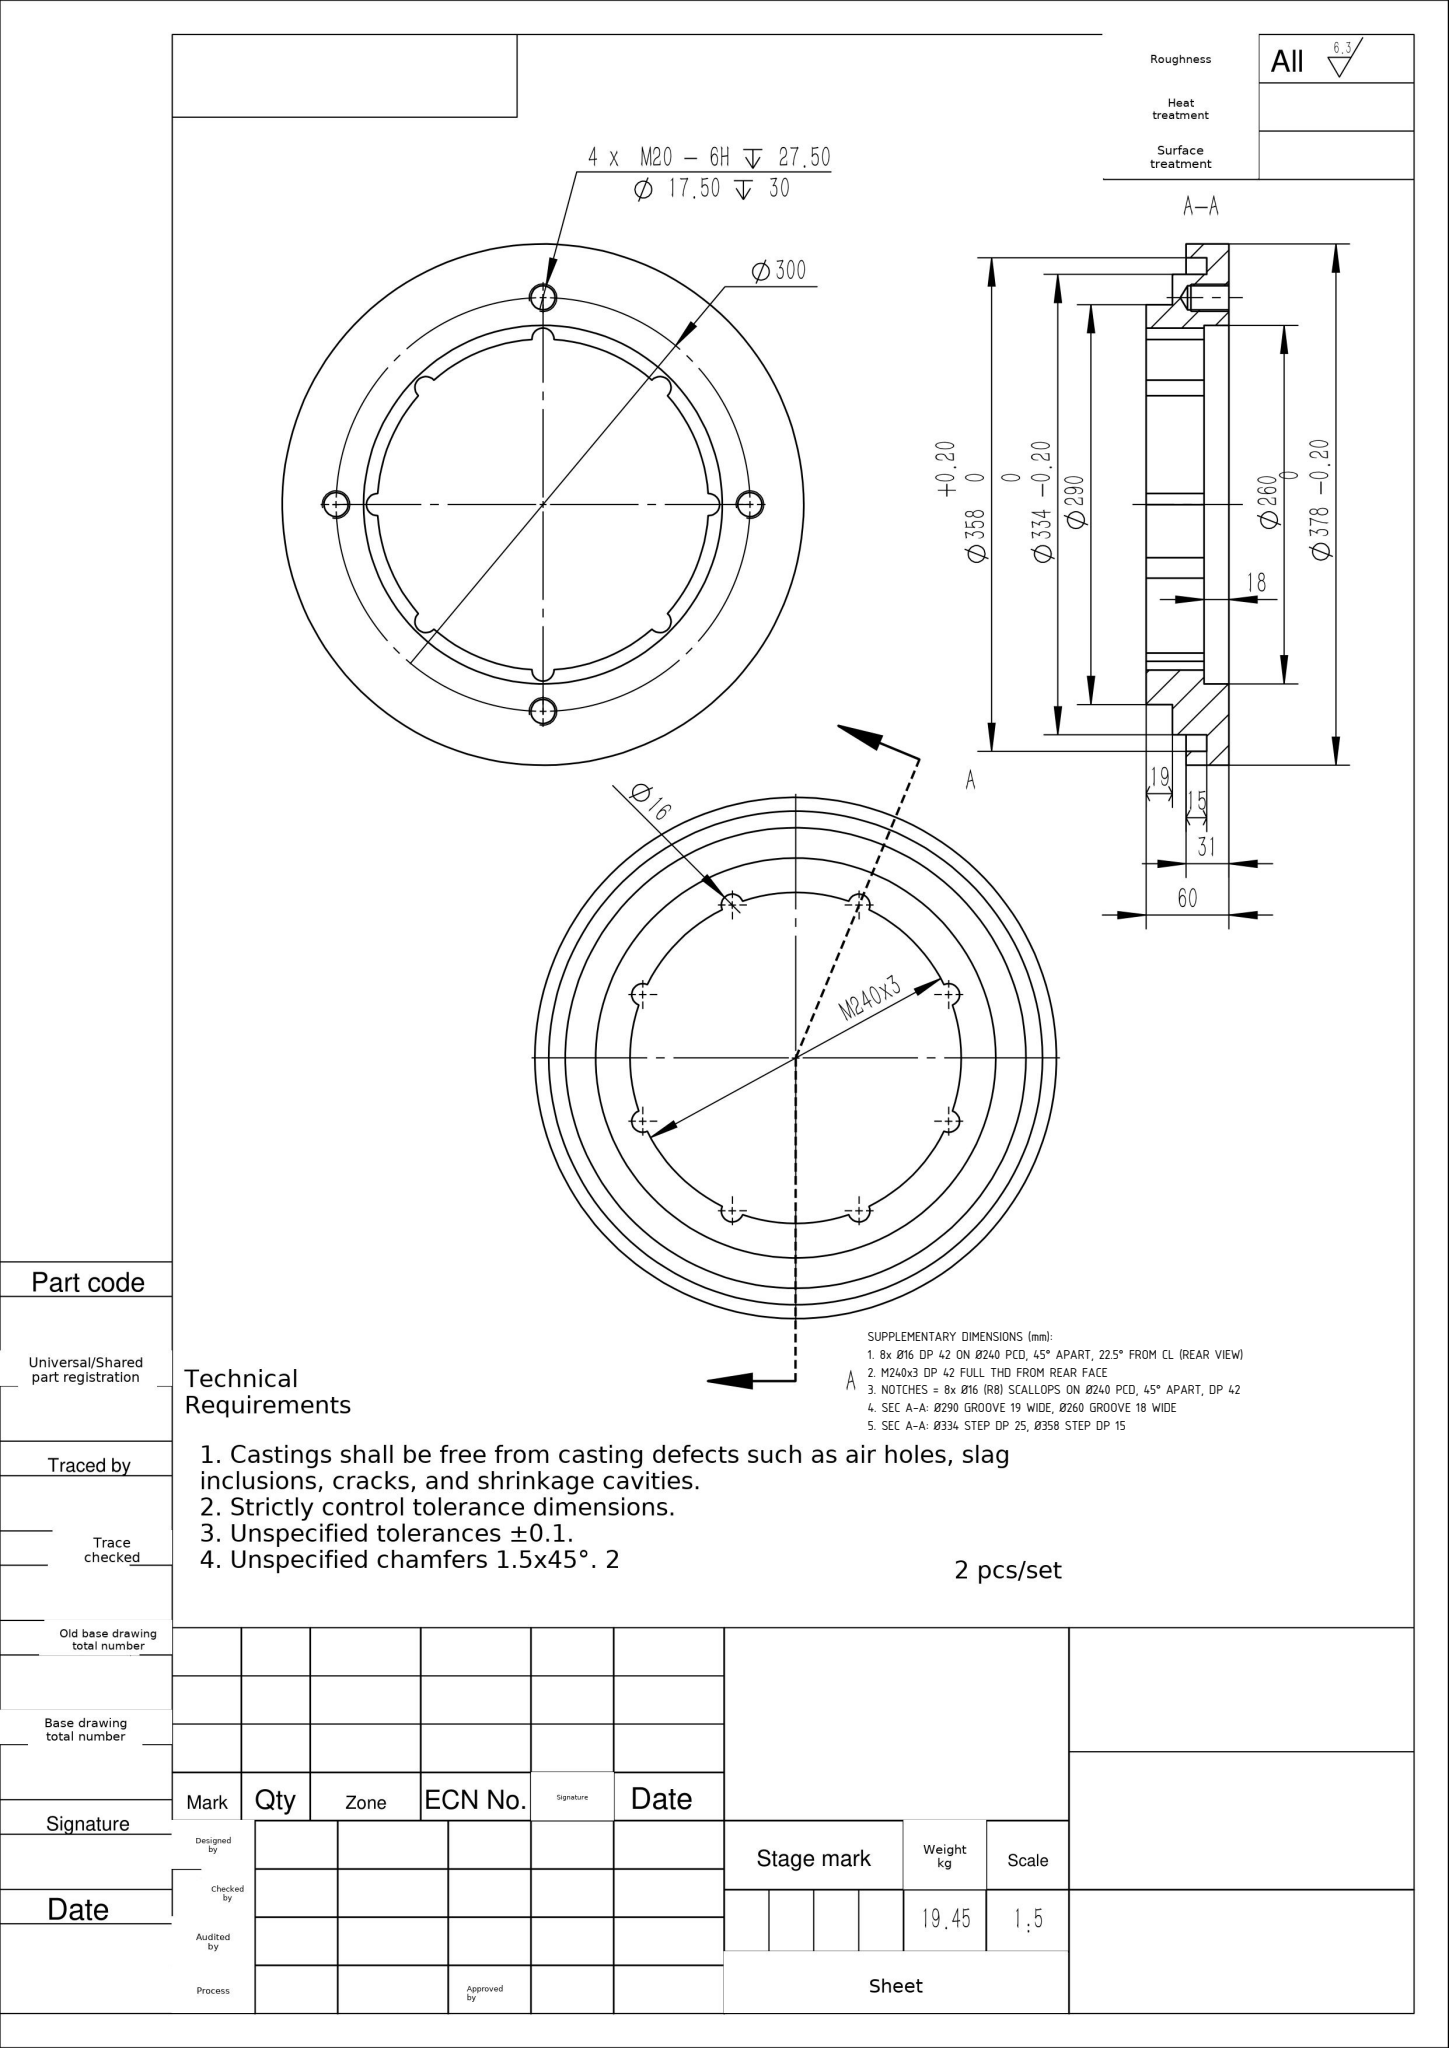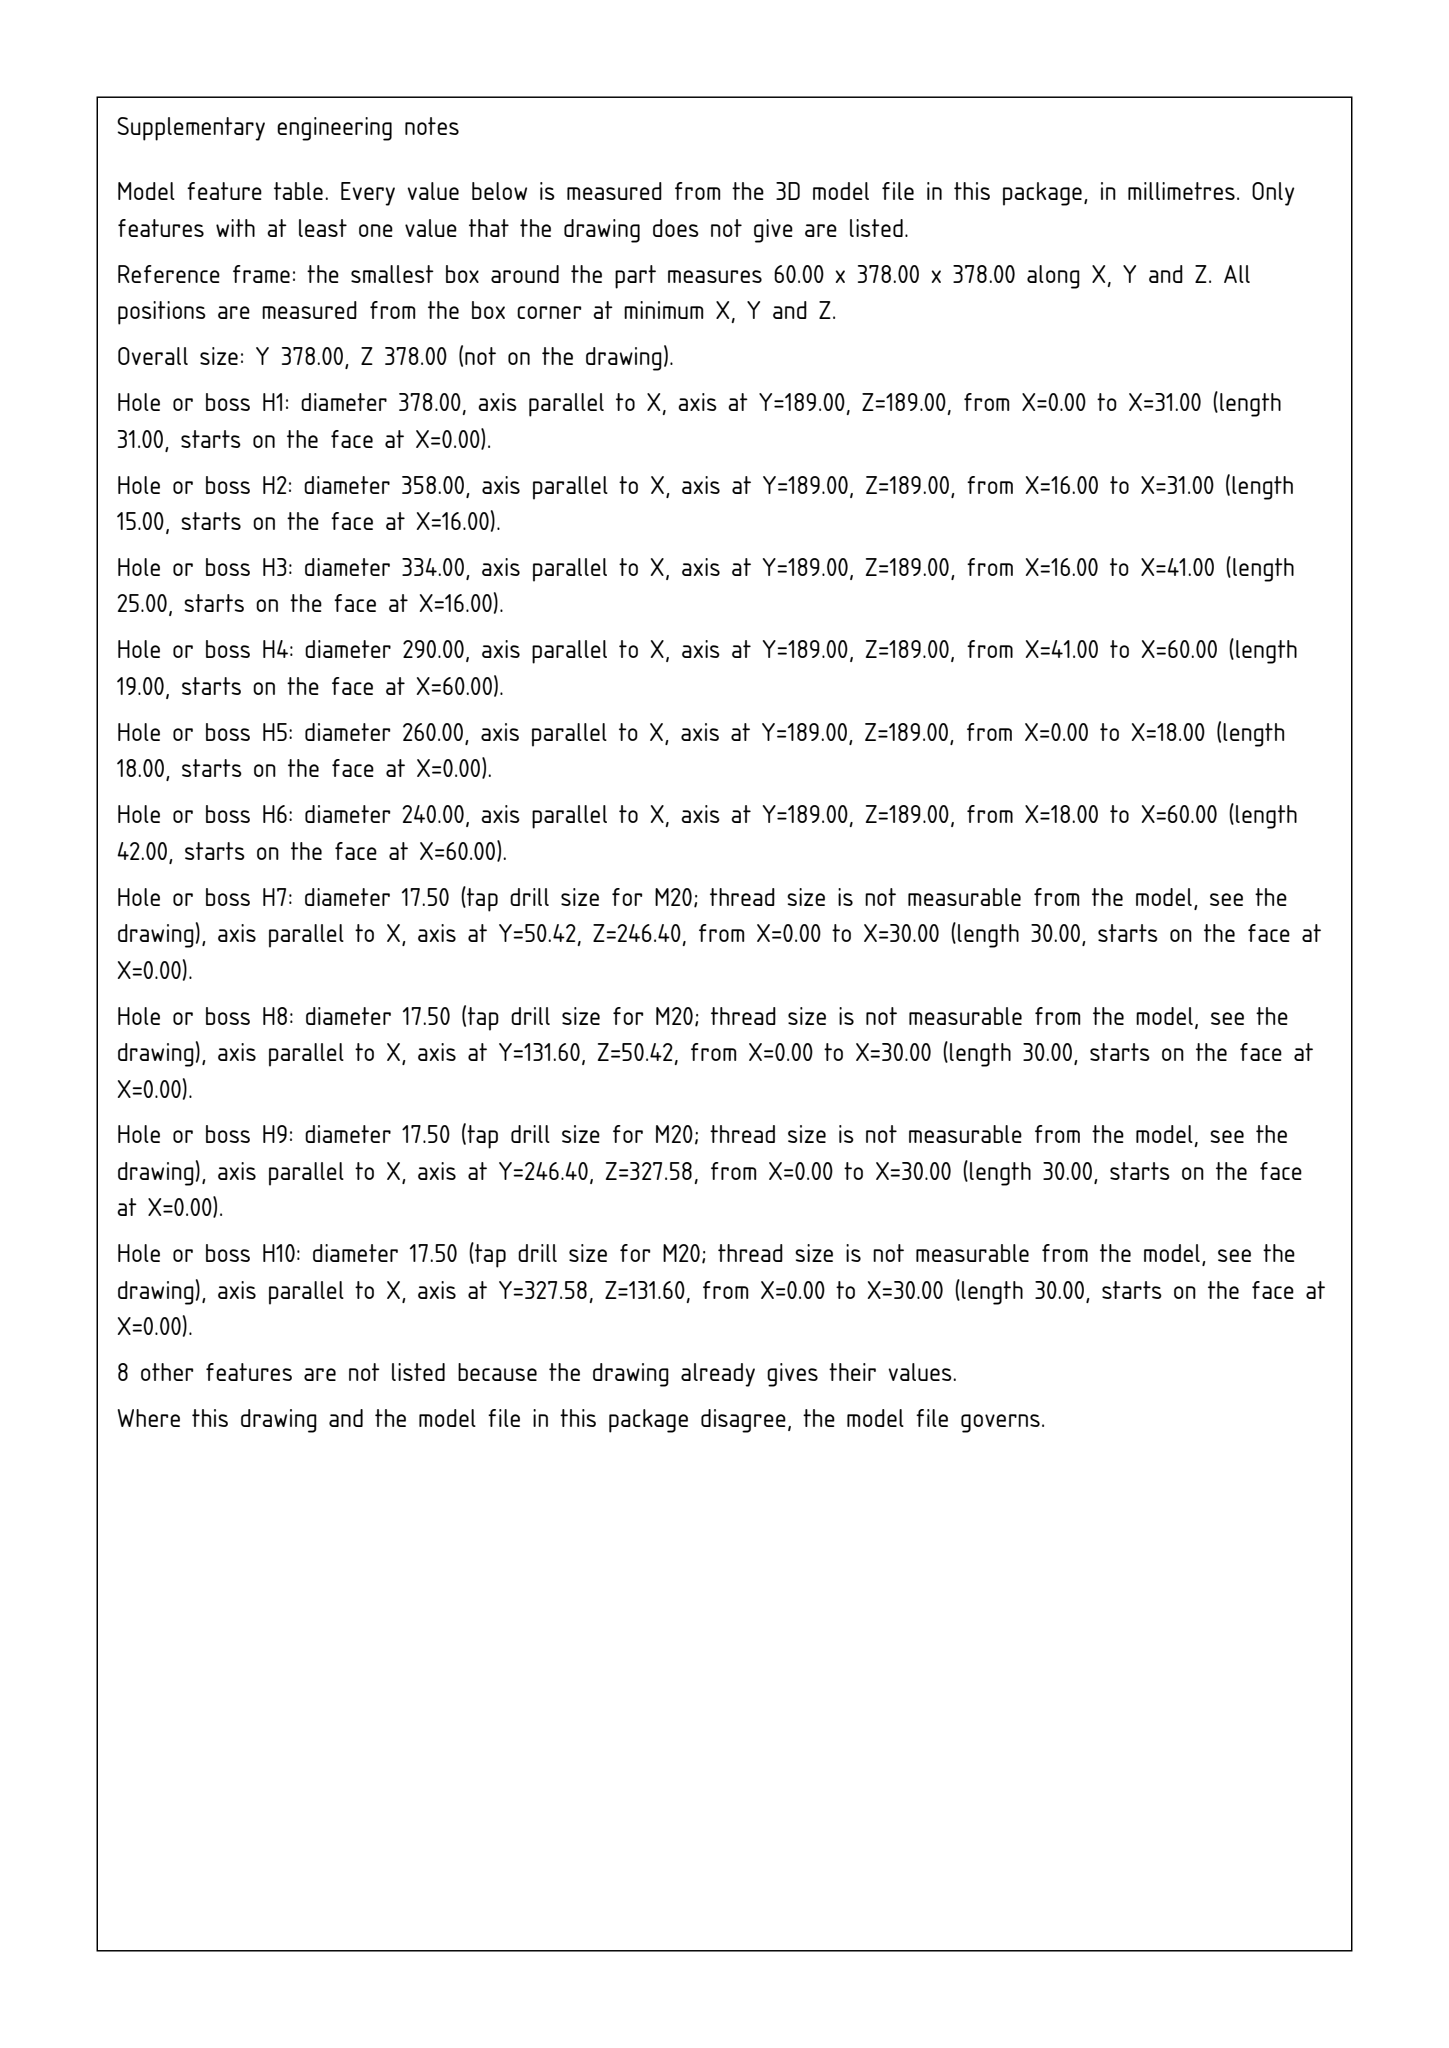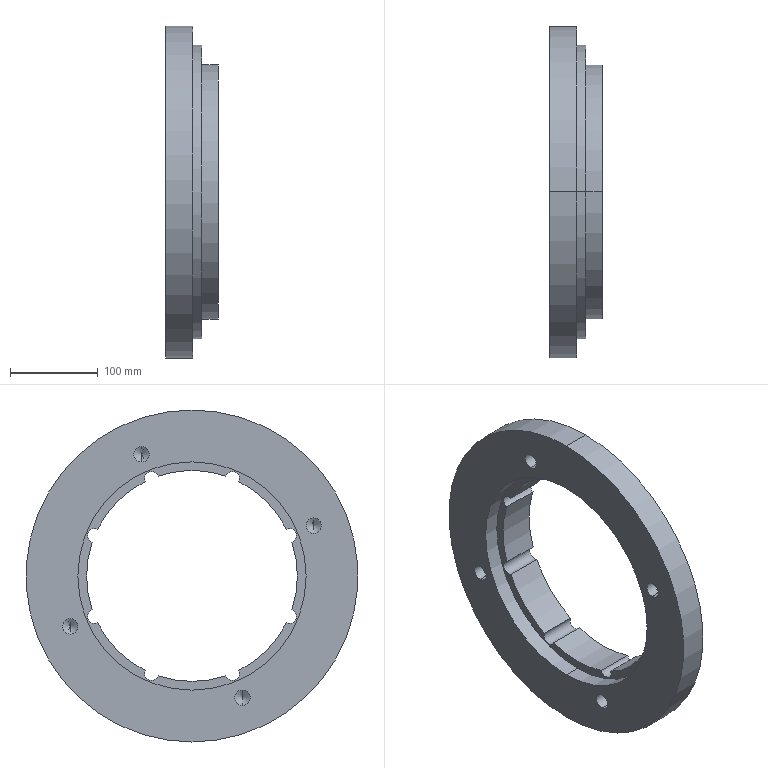Part | SolidWorks | mm | 1 solid | 49 faces | box 60 x 378 x 378 mm | volume 2493820 mm3 | cylinder 35 | cone 8 | plane 6 | commonest cylinder face diameters 240 x9 17.5 x8 16 x8 260 x2 290 x2 334 x2 358 x2 378 x2
build123d program:
from build123d import *

# Parameters (mm, degrees)
BOSS_EXTRUDE1_START = 30
SKETCH2_R           = 162.447
SKETCH2_R_2         = 120
BOSS_EXTRUDE1_DEPTH = 30
SKETCH3_R           = 145
SKETCH3_R_2         = 120
BOSS_EXTRUDE2_DEPTH = 29
SKETCH4_R           = 167
SKETCH4_R_2         = 145
BOSS_EXTRUDE3_DEPTH = 10
SKETCH5_R           = 176.563
CUT_EXTRUDE1_DEPTH  = 30
SKETCH6_R           = 135
CUT_EXTRUDE2_DEPTH  = 15
SKETCH7_R           = 8
CUT_EXTRUDE3_DEPTH  = 65
CIRPATTERN1_COUNT   = 8
BOSS_EXTRUDE4_START = 3
SKETCH8_R           = 190
SKETCH8_R_2         = 135
BOSS_EXTRUDE4_DEPTH = 3
BOSS_EXTRUDE6_START = 18
SKETCH12_R          = 135
SKETCH12_R_2        = 130
BOSS_EXTRUDE6_DEPTH = 18
CIRPATTERN2_COUNT   = 4
SKETCH15_R          = 209.769
SKETCH15_R_2        = 189
CUT_EXTRUDE6_DEPTH  = 30


with BuildPart() as part:
    # Sketch1 → Revolve1 (revolve)
    with BuildSketch(Plane.XY, mode=Mode.PRIVATE) as revolve1_sk:
        Polygon((-47, 189), (-19, 189), (-19, 179), (-34, 179), (-34, 167), (-19, 167), (-19, 120), (-47, 120), align=None)
    revolve(revolve1_sk.sketch.rotate(Axis((-53.36, 0, 0), (1, 0, 0)), 90), axis=Axis((-53.36, 0, 0), (1, 0, 0)))

    # Sketch2 → Boss-Extrude1 (add)
    with BuildSketch(Plane.ZY.offset(47).offset(BOSS_EXTRUDE1_START)):
        with Locations(Location((0, 0, 0), (0, 0, 180))):
            Circle(SKETCH2_R)
        Circle(SKETCH2_R_2, mode=Mode.SUBTRACT)
    extrude(amount=-BOSS_EXTRUDE1_DEPTH)

    # Sketch3 → Boss-Extrude2 (add)
    with BuildSketch(Plane(origin=(-19, 0, 0), x_dir=(0, 0, -1), z_dir=(1, 0, 0))):
        with Locations(Location((0, 0, 0), (0, 0, 180))):
            Circle(SKETCH3_R)
        with Locations(Location((0, 0, 0), (0, 0, 180))):
            Circle(SKETCH3_R_2, mode=Mode.SUBTRACT)
    extrude(amount=BOSS_EXTRUDE2_DEPTH)

    # Sketch4 → Boss-Extrude3 (add)
    with BuildSketch(Plane(origin=(-19, 0, 0), x_dir=(0, 0, -1), z_dir=(1, 0, 0))):
        with Locations(Location((0, 0, 0), (0, 0, 180))):
            Circle(SKETCH4_R)
        with Locations(Location((0, 0, 0), (0, 0, 180))):
            Circle(SKETCH4_R_2, mode=Mode.SUBTRACT)
    extrude(amount=BOSS_EXTRUDE3_DEPTH)

    # Sketch5 → Cut-Extrude1 (cut)
    with BuildSketch(Plane.ZY.offset(77)):
        Circle(SKETCH5_R)
    extrude(amount=-CUT_EXTRUDE1_DEPTH, mode=Mode.SUBTRACT)

    # Sketch6 → Cut-Extrude2 (cut)
    with BuildSketch(Plane.ZY.offset(47)):
        Circle(SKETCH6_R)
    extrude(amount=-CUT_EXTRUDE2_DEPTH, mode=Mode.SUBTRACT)

    # Sketch7 → Cut-Extrude3 (cut)
    with BuildSketch(Plane.ZY.offset(32)):
        with Locations((-45.922, 110.866)):
            Circle(SKETCH7_R)
    cut_extrude3 = extrude(amount=-CUT_EXTRUDE3_DEPTH, mode=Mode.SUBTRACT)

    # CirPattern1: Cut-Extrude3 ×8 about axis
    cirpattern1_axis = Axis((0, 0, 0), (1, 0, 0))
    for i in range(1, CIRPATTERN1_COUNT):
        add(cut_extrude3.rotate(cirpattern1_axis, i * 360 / CIRPATTERN1_COUNT), mode=Mode.SUBTRACT)

    # Sketch8 → Boss-Extrude4 (add)
    with BuildSketch(Plane.ZY.offset(47).offset(BOSS_EXTRUDE4_START)):
        Circle(SKETCH8_R)
        Circle(SKETCH8_R_2, mode=Mode.SUBTRACT)
    extrude(amount=-BOSS_EXTRUDE4_DEPTH)

    # Sketch12 → Boss-Extrude6 (add)
    with BuildSketch(Plane.ZY.offset(32).offset(BOSS_EXTRUDE6_START)):
        Circle(SKETCH12_R)
        Circle(SKETCH12_R_2, mode=Mode.SUBTRACT)
    extrude(amount=-BOSS_EXTRUDE6_DEPTH)

    # Sketch17 → M20 Tapped Hole1 (revolve, cut)
    with BuildSketch(Plane(origin=(-50, 138.582, -57.403), x_dir=(0, 0, 1), z_dir=(0, 1, 0))):
        Polygon((0, 0), (0, 35.258), (8.75, 30), (8.75, 0), align=None)
    m20_tapped_hole1 = revolve(axis=Axis((-56.35, 138.582, -57.403), (1, 0, 0)), mode=Mode.SUBTRACT)

    # CirPattern2: M20 Tapped Hole1 ×4 about axis
    cirpattern2_axis = Axis((0, 0, 0), (1, 0, 0))
    for i in range(1, CIRPATTERN2_COUNT):
        add(m20_tapped_hole1.rotate(cirpattern2_axis, i * 360 / CIRPATTERN2_COUNT), mode=Mode.SUBTRACT)

    # Sketch15 → Cut-Extrude6 (cut)
    with BuildSketch(Plane(origin=(-47, 0, 0), x_dir=(0, 0, -1), z_dir=(1, 0, 0))):
        Circle(SKETCH15_R)
        with Locations(Location((0, 0, 0), (0, 0, 180))):
            Circle(SKETCH15_R_2, mode=Mode.SUBTRACT)
    extrude(amount=-CUT_EXTRUDE6_DEPTH, mode=Mode.SUBTRACT)


solid = part.part